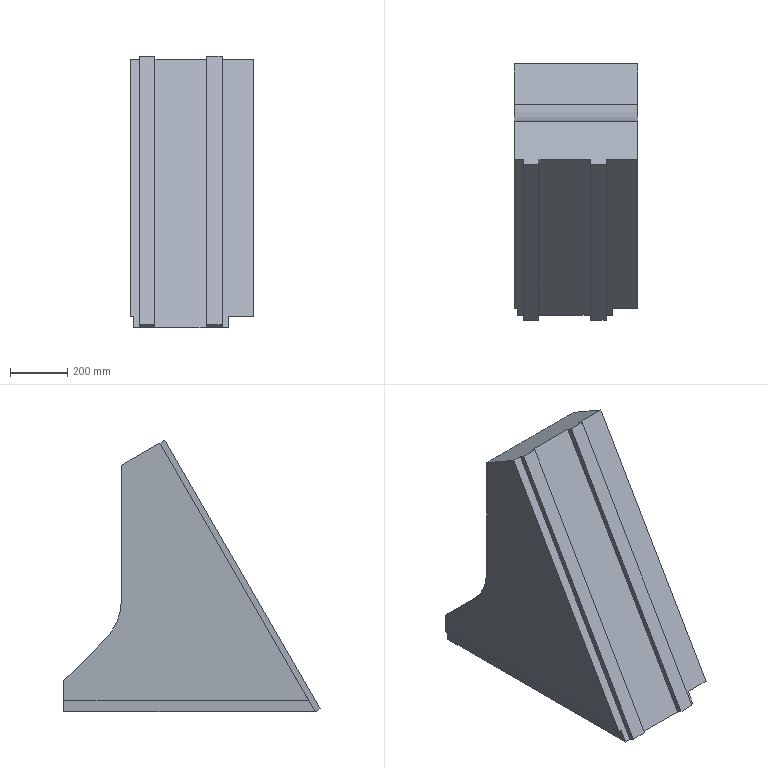Component | NX | SIM15_Y1_SCHLITTEN | 1 solid | 21 faces | volume 178346655 mm3 | plane 20 | cylinder 1 | commonest cylinder face diameters 400 x1